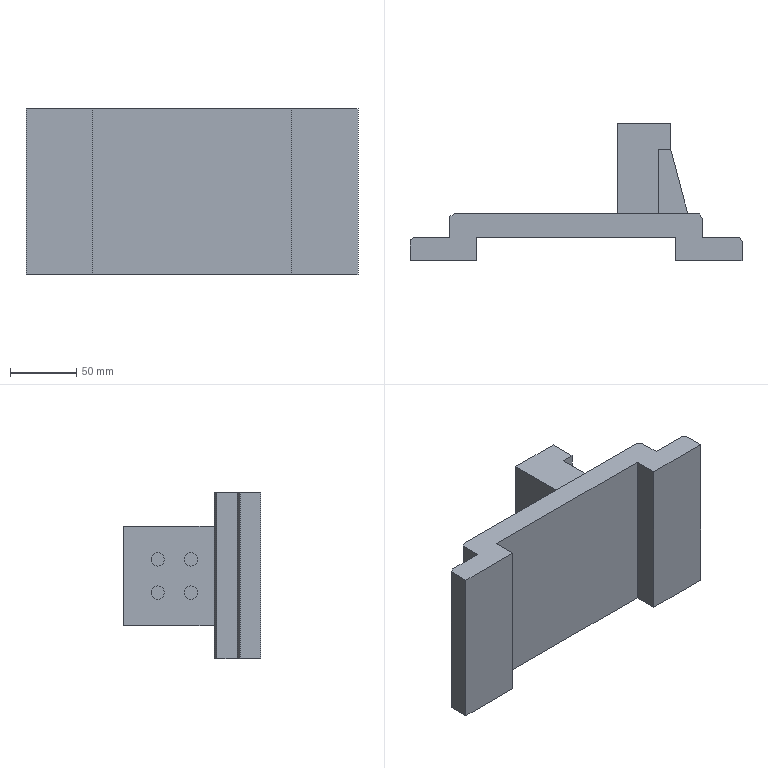Component | NX | JIG_BODY | 1 solid | 48 faces | volume 827680 mm3 | plane 35 | cylinder 9 | cone 4 | commonest cylinder face diameters 10 x8 12 x1